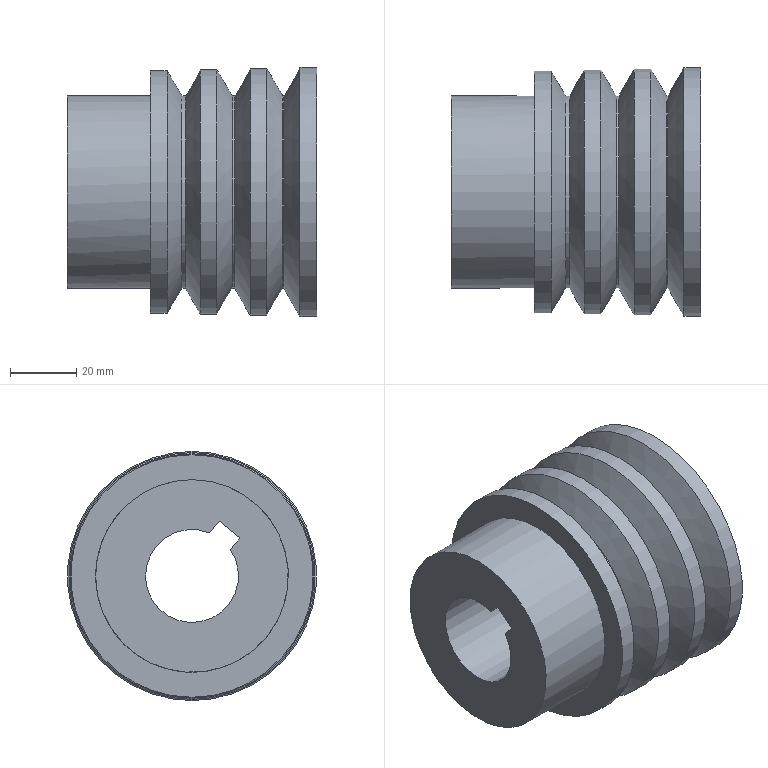Component | NX | SMALL_PULLEY | 1 solid | 21 faces | volume 204530 mm3 | cylinder 9 | plane 6 | cone 6 | commonest cylinder face diameters 58 x4 28 x1 73.01 x1 75 x1 73.575 x1 74.287 x1